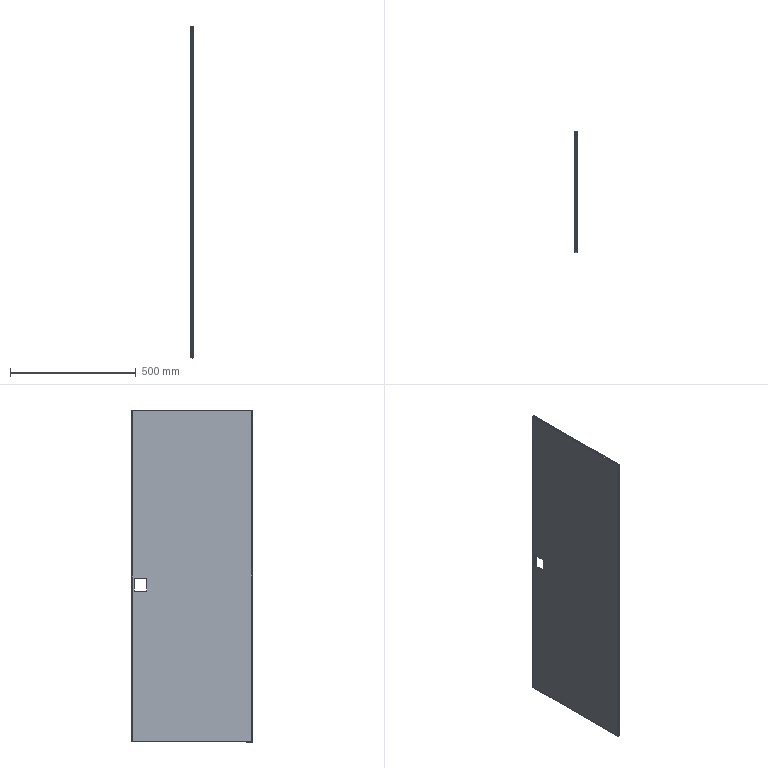Component | SolidWorks | RightDoor-1 | 1 solid | 76 faces | volume 1027612 mm3 | plane 44 | spline 16 | cylinder 16 | commonest cylinder face diameters 5 x8 2 x8